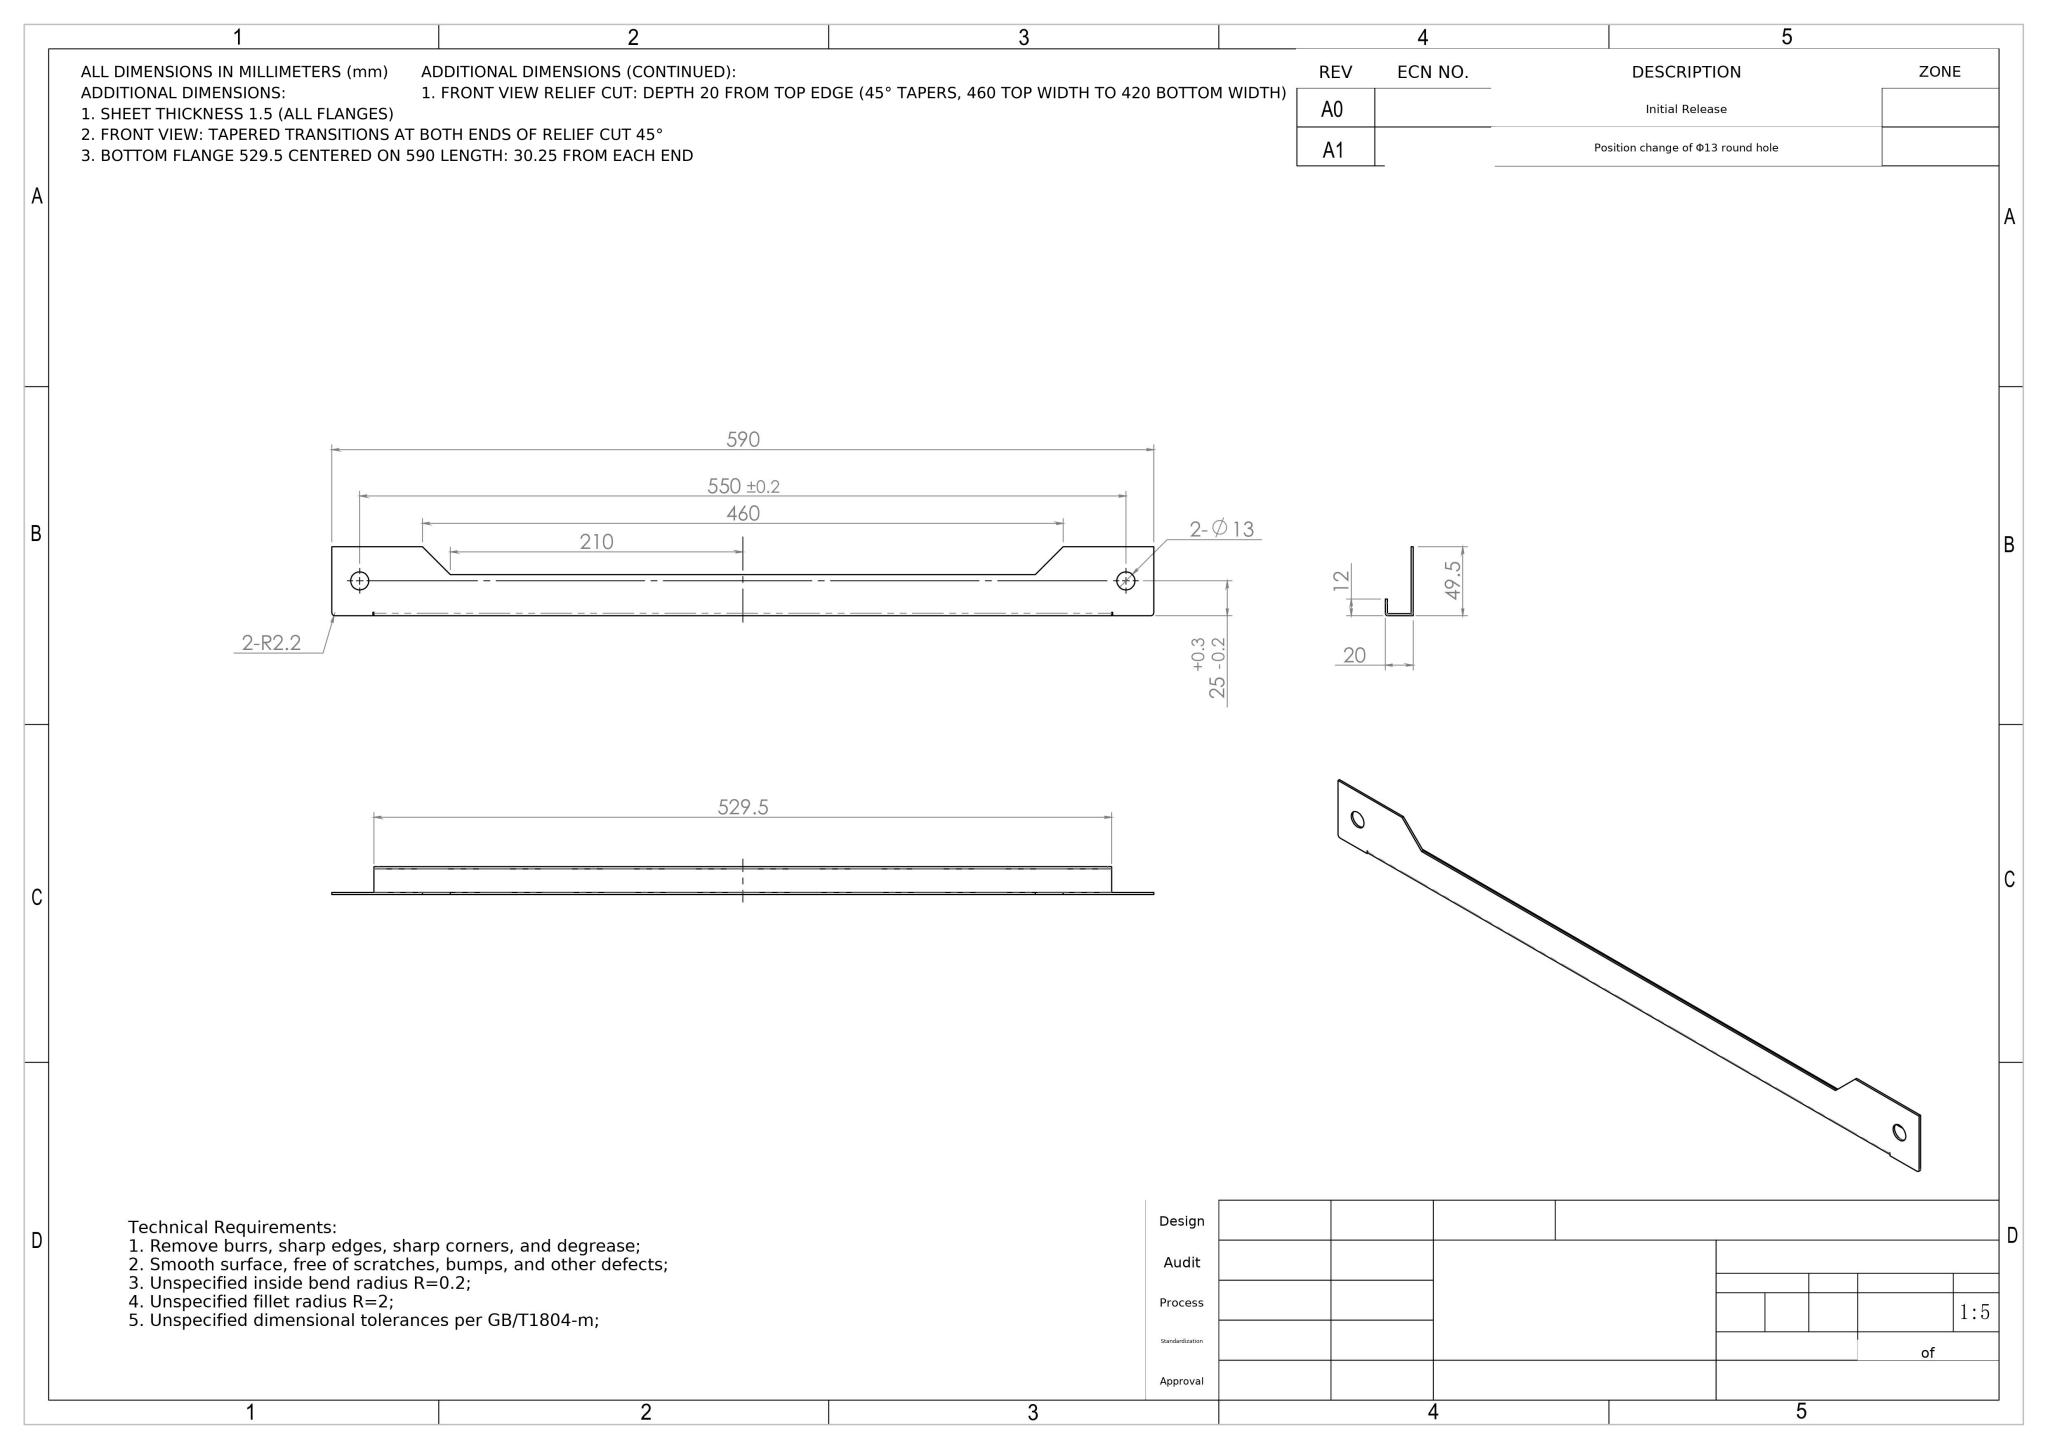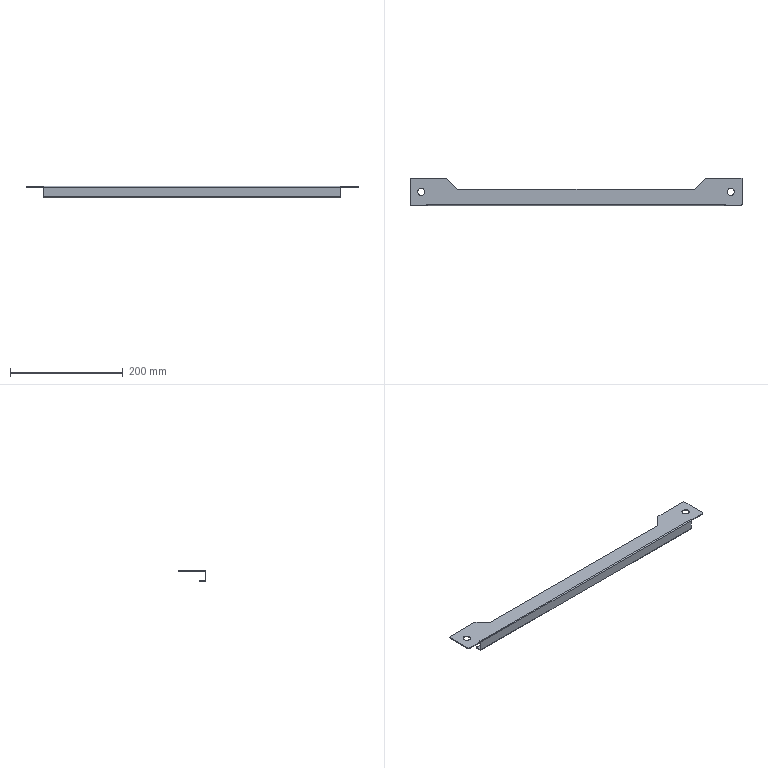Part | NX | mm | 1 solid | 42 faces | box 590 x 49.5 x 20 mm | volume 52580 mm3 | plane 30 | cylinder 12 | commonest cylinder face diameters 13 x4 3.4 x2 0.4 x2 6 x2 4.4 x2